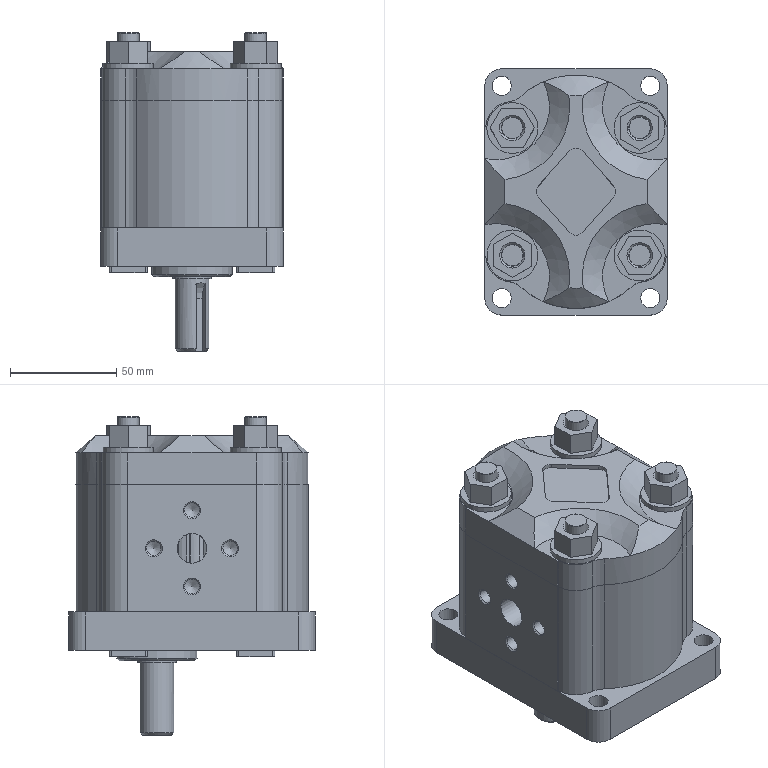Assembly | NX | mm | 33 component files | 33 solids | 774 faces | box 86 x 116 x 149.9 mm | volume 747480 mm3 | plane 360 | cylinder 248 | spline 55 | other 55 | cone 54 | torus 2 | commonest cylinder face diameters 2 x24 20 x16 18 x16 39 x13 24 x12 13 x12 12.5 x12 25.4 x11
Bill of materials:
CLYF-12 | 2 |  | Thin flat clip with a double-C (figure-eight) outline: two open C-shaped arcs joined at a narrow central neck, each arc ending in a short angled tab.
GB/T 97.1-2002 | 4 |  | Flat annular disc (plain washer shape) with a concentric through-hole.
CLYF-03 | 1 |  | Stepped cylindrical shaft with an integral spur pinion (about 11-12 teeth) near one end and a slot or flat near the other end.
CLYF-06 | 1 |  | Thick plate or cover with a lobed, roughly rectangular outline, four corner through-holes, and curved scalloped recesses between the hole bosses on one face.
GB/T8-1988 | 4 |  | Stepped cylindrical pin rising from a square base block with rounded corners.
GB/T 6170-2000 | 4 |  | Hexagonal prism (nut-like body) with a central cylindrical through-bore that has a chamfer or countersink at the opening.
GB/T 119.1-2000 | 2 |  | Solid-looking right circular cylinder with a small chamfer around both end edges and flat end faces; length is roughly 1.5 times the diameter.
CLYB-13 | 2 |  | Thin flat obround (stadium-shaped) closed loop with a narrow, uniform band width.
CLYF-02 | 1 |  | Block-shaped housing with a lobed outline, a figure-eight (two overlapping circles) through-cavity, a groove around the cavity, four corner through-holes, and a side port surrounded by four blind holes.
CLYF-01 | 1 |  | Rectangular plate with rounded corners and multiple holes, plus a short cylindrical chamfered boss on the underside.
CLYF-05 | 2 |  | Figure-eight block with two parallel through-bores, interrupted annular recesses around each bore on one face, and semicircular notches at the waist.
GB/T 983.1-1986 | 1 |  | Thin flat split ring with two ends that have small circular holes in lug tabs, with the lugs on the inner side of the ring.
CLYF-15 | 1 |  | Thick plain annular ring (spacer/bushing shape) with a concentric through-bore.
CLYF-07 | 2 |  | Thin-walled hollow cylinder (tube/sleeve) with open ends; length is roughly equal to its outer diameter.
GB/T 93-1987 | 4 |  | Flat annular ring (washer- or spacer-like) with a concentric central through hole, a wide radial face and a short axial thickness.
CLYF-04 | 1 |  | Small spur pinion made in one piece with a straight cylindrical shaft. The toothed section is roughly mid-length, and the shaft sticks out on both sides with chamfered ends.
Mates:
1. fix | 2 1 component
2. touch align | 5 2 face | 2 1 face
3. touch align | 5 2 face | 2 1 face
4. touch align | 5 2 face | 2 1 face
5. touch align | 12 2 face | 5 2 face
6. touch align | 12 2 face | 5 2 face
7. touch align | 12 2 face | 5 2 face
8. touch align | 13 2 face | 5 2 face
9. touch align | 13 2 face | 5 2 face
10. touch align | 13 2 face | 2 1 face
11. touch align | 3 1 face | 5 2 face
12. touch align | 3 1 face | 5 2 face
13. touch align | 4 1 face | 5 2 face
14. touch align | 4 1 face | 5 2 face
15. touch align | 7 2 face | 4 1 face
16. touch align | 7 2 face | 4 1 face
17. touch align | 6 1 face | 2 1 face
18. touch align | 6 1 face | 2 1 face
19. touch align | 6 1 face | 2 1 face
20. touch align | 9 4 face | 2 1 face
21. touch align | 9 4 face | 10 4 face
22. touch align | 11 4 face | 6 1 face
23. touch align | 8 4 face | 9 4 face
24. touch align | 8 4 face | 11 4 face
25. fix | assembly component
26. bond | 10 4 component | assembly component
27. bond | 8 4 component | assembly component
28. bond | 11 4 component | assembly component
29. bond | 9 4 component | assembly component
30. bond | 10 3 component | assembly component
31. bond | 8 3 component | assembly component
32. bond | 11 3 component | assembly component
33. bond | 9 3 component | assembly component
34. bond | 10 2 component | assembly component
35. bond | 8 2 component | assembly component
36. bond | 11 2 component | assembly component
37. bond | 9 2 component | assembly component
38. circular | assembly datumaxis | assembly cartesiancoordinatesystem | assembly cartesiancoordinatesystem | assembly cartesiancoordinatesystem | assembly cartesiancoordinatesystem
39. circular | assembly datumaxis | assembly cartesiancoordinatesystem | assembly cartesiancoordinatesystem | assembly cartesiancoordinatesystem | assembly cartesiancoordinatesystem
40. circular | assembly datumaxis | assembly cartesiancoordinatesystem | assembly cartesiancoordinatesystem | assembly cartesiancoordinatesystem | assembly cartesiancoordinatesystem
41. circular | assembly datumaxis | assembly cartesiancoordinatesystem | assembly cartesiancoordinatesystem | assembly cartesiancoordinatesystem | assembly cartesiancoordinatesystem
42. bond | 10 1 component | assembly component
43. bond | 8 1 component | assembly component
44. bond | 11 1 component | assembly component
45. bond | 9 1 component | assembly component
46. touch align | 14 2 face | 2 1 face
47. touch align | 14 1 face | 2 1 face
48. touch align | 1 1 face | 3 1 face
49. touch align | 1 1 face | 14 2 face
50. touch align | 1 1 face | 2 1 face
51. touch align | 10 4 face | 1 1 face
52. touch align | 16 1 face | 1 1 face
53. touch align | 16 1 face | 1 1 face
54. touch align | 15 1 face | 1 1 face
55. touch align | 15 1 face | 1 1 face
56. distance | 14 1 face | 2 1 face
57. distance | 14 2 face | 2 1 face
58. touch align | 11 4 face | 9 4 face